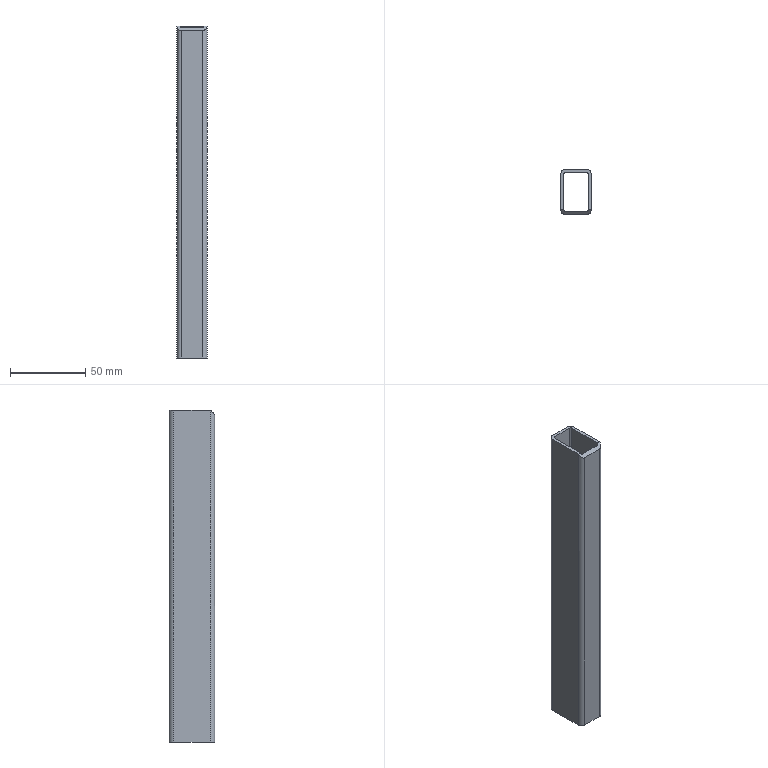Component | SolidWorks | A30x20x2RectangularColdFormedHollowSectionSteel220-1 | 1 solid | 19 faces | box 20 x 30 x 220 mm | volume 38896 mm3 | plane 11 | cylinder 8 | commonest cylinder face diameters 6 x4 2 x4
build123d program:
from build123d import *

# Parameters (mm, degrees)
BOSS_EXTRUDE1_DEPTH     = 220
CUT_EXTRUDE1_DEPTH      = 221.737
CUT_EXTRUDE1_DEPTH_BACK = 221.737


with BuildPart() as part:
    # Sketch1_2 → Boss-Extrude1 (new body)
    with BuildSketch(Plane(origin=(0, 0, 0), x_dir=(0, 0, -1), z_dir=(1, 0, 0))):
        with BuildLine():
            Line((-6.263, 13), (6.263, 13))
            Line((6.263, 13), (7.561, 14.947))
            ThreePointArc((7.561, 14.947), (7.282, 14.987), (7, 15))
            Line((7, 15), (-7, 15))
            ThreePointArc((-7, 15), (-7.282, 14.987), (-7.561, 14.947))
            Line((-7.561, 14.947), (-6.263, 13))
        make_face()
        with BuildLine():
            Line((-10, -11.394), (-8, -8.394))
            Line((-8, -8.394), (-8, 12))
            ThreePointArc((-8, 12), (-7.707, 12.707), (-7, 13))
            Line((-7, 13), (-6.263, 13))
            Line((-6.263, 13), (-7.561, 14.947))
            ThreePointArc((-7.561, 14.947), (-9.311, 13.913), (-10, 12))
            Line((-10, 12), (-10, -11.394))
        make_face()
        with BuildLine():
            Line((8, 12), (8, -8.394))
            Line((8, -8.394), (10, -11.394))
            Line((10, -11.394), (10, 12))
            ThreePointArc((10, 12), (9.311, 13.913), (7.561, 14.947))
            Line((7.561, 14.947), (6.263, 13))
            Line((6.263, 13), (7, 13))
            ThreePointArc((7, 13), (7.707, 12.707), (8, 12))
        make_face()
        with BuildLine():
            Line((7, -13), (-7, -13))
            ThreePointArc((-7, -13), (-7.707, -12.707), (-8, -12))
            Line((-8, -12), (-8, -8.394))
            Line((-8, -8.394), (-10, -11.394))
            Line((-10, -11.394), (-10, -12))
            ThreePointArc((-10, -12), (-9.121, -14.121), (-7, -15))
            Line((-7, -15), (7, -15))
            ThreePointArc((7, -15), (9.121, -14.121), (10, -12))
            Line((10, -12), (10, -11.394))
            Line((10, -11.394), (8, -8.394))
            Line((8, -8.394), (8, -12))
            ThreePointArc((8, -12), (7.707, -12.707), (7, -13))
        make_face()
    extrude(amount=BOSS_EXTRUDE1_DEPTH)

    # Sketch1 → Cut-Extrude1 (cut, two sides: drawn at the far end of the back side and taken through both)
    with BuildSketch(Plane.XY.offset(-CUT_EXTRUDE1_DEPTH_BACK)):
        Polygon((221, 11), (221, 16), (216, 16), align=None)
    extrude(amount=CUT_EXTRUDE1_DEPTH + CUT_EXTRUDE1_DEPTH_BACK, mode=Mode.SUBTRACT)


solid = part.part

# Placed as in the assembly
solid = solid.moved(Location((-452.371, -1060.9, 193), (180, 90, 0)))
STEP:
#1=COLOUR_RGB('',0.7922,0.8196,0.9333);
#2=FILL_AREA_STYLE_COLOUR('',#1);
#3=FILL_AREA_STYLE('',(#2));
#4=SURFACE_STYLE_FILL_AREA(#3);
#5=SURFACE_SIDE_STYLE('',(#4));
#6=SURFACE_STYLE_USAGE(.BOTH.,#5);
#7=PRESENTATION_STYLE_ASSIGNMENT((#6));
#8=CARTESIAN_POINT('',(-17.534,-42.358,16.142));
#9=VERTEX_POINT('',#8);
#10=CARTESIAN_POINT('',(-17.416,-42.24,16.26));
#11=VERTEX_POINT('',#10);
#12=CARTESIAN_POINT('',(-17.534,-42.358,16.142));
#13=CARTESIAN_POINT('',(-17.465,-42.358,16.142));
#14=CARTESIAN_POINT('',(-17.416,-42.309,16.191));
#15=CARTESIAN_POINT('',(-17.416,-42.24,16.26));
#16=(BOUNDED_CURVE()B_SPLINE_CURVE(3,(#12,#13,#14,#15),.UNSPECIFIED.,.F.,.T.)B_SPLINE_CURVE_WITH_KNOTS((4,4),(0.,1.571),.UNSPECIFIED.)CURVE()GEOMETRIC_REPRESENTATION_ITEM()RATIONAL_B_SPLINE_CURVE((1.,0.8047,0.8047,1.))REPRESENTATION_ITEM(''));
#17=EDGE_CURVE('',#9,#11,#16,.T.);
#18=ORIENTED_EDGE('',*,*,#17,.F.);
#19=CARTESIAN_POINT('',(-17.534,-42.358,7.598));
#20=VERTEX_POINT('',#19);
#21=CARTESIAN_POINT('',(-17.534,-42.358,16.26));
#22=DIRECTION('',(0.,0.,-1.));
#23=VECTOR('',#22,39.37);
#24=LINE('',#21,#23);
#25=EDGE_CURVE('',#9,#20,#24,.T.);
#26=ORIENTED_EDGE('',*,*,#25,.T.);
#27=CARTESIAN_POINT('',(-17.416,-42.24,7.598));
#28=VERTEX_POINT('',#27);
#29=CARTESIAN_POINT('',(-17.534,-42.24,7.598));
#30=DIRECTION('',(0.,0.,-1.));
#31=DIRECTION('',(-1.,0.,0.));
#32=AXIS2_PLACEMENT_3D('',#29,#30,#31);
#33=CIRCLE('',#32,0.1181);
#34=EDGE_CURVE('',#28,#20,#33,.T.);
#35=ORIENTED_EDGE('',*,*,#34,.F.);
#36=CARTESIAN_POINT('',(-17.416,-42.24,16.26));
#37=DIRECTION('',(0.,0.,-1.));
#38=VECTOR('',#37,39.37);
#39=LINE('',#36,#38);
#40=EDGE_CURVE('',#11,#28,#39,.T.);
#41=ORIENTED_EDGE('',*,*,#40,.F.);
#42=EDGE_LOOP('',(#18,#26,#35,#41));
#43=FACE_OUTER_BOUND('',#42,.T.);
#44=CARTESIAN_POINT('',(-17.534,-42.24,16.26));
#45=DIRECTION('',(0.,0.,-1.));
#46=DIRECTION('',(1.,0.,0.));
#47=AXIS2_PLACEMENT_3D('',#44,#45,#46);
#48=CYLINDRICAL_SURFACE('',#47,0.1181);
#49=ADVANCED_FACE('',(#43),#48,.T.);
#50=CARTESIAN_POINT('',(-17.416,-41.295,7.598));
#51=VERTEX_POINT('',#50);
#52=CARTESIAN_POINT('',(-17.416,-41.768,7.598));
#53=DIRECTION('',(0.,-1.,-0.));
#54=VECTOR('',#53,39.37);
#55=LINE('',#52,#54);
#56=EDGE_CURVE('',#51,#28,#55,.T.);
#57=ORIENTED_EDGE('',*,*,#56,.F.);
#58=CARTESIAN_POINT('',(-17.416,-41.295,16.26));
#59=VERTEX_POINT('',#58);
#60=CARTESIAN_POINT('',(-17.416,-41.295,16.26));
#61=DIRECTION('',(0.,0.,-1.));
#62=VECTOR('',#61,39.37);
#63=LINE('',#60,#62);
#64=EDGE_CURVE('',#59,#51,#63,.T.);
#65=ORIENTED_EDGE('',*,*,#64,.F.);
#66=CARTESIAN_POINT('',(-17.416,-41.768,16.26));
#67=DIRECTION('',(0.,-1.,-0.));
#68=VECTOR('',#67,39.37);
#69=LINE('',#66,#68);
#70=EDGE_CURVE('',#59,#11,#69,.T.);
#71=ORIENTED_EDGE('',*,*,#70,.T.);
#72=ORIENTED_EDGE('',*,*,#40,.T.);
#73=EDGE_LOOP('',(#57,#65,#71,#72));
#74=FACE_OUTER_BOUND('',#73,.T.);
#75=CARTESIAN_POINT('',(-17.416,-41.768,16.26));
#76=DIRECTION('',(1.,0.,0.));
#77=DIRECTION('',(-0.,-0.,1.));
#78=AXIS2_PLACEMENT_3D('',#75,#76,#77);
#79=PLANE('',#78);
#80=ADVANCED_FACE('',(#74),#79,.T.);
#81=CARTESIAN_POINT('',(-17.534,-41.177,7.598));
#82=VERTEX_POINT('',#81);
#83=CARTESIAN_POINT('',(-17.534,-41.295,7.598));
#84=DIRECTION('',(0.,0.,-1.));
#85=DIRECTION('',(-1.,0.,0.));
#86=AXIS2_PLACEMENT_3D('',#83,#84,#85);
#87=CIRCLE('',#86,0.1181);
#88=EDGE_CURVE('',#82,#51,#87,.T.);
#89=ORIENTED_EDGE('',*,*,#88,.F.);
#90=CARTESIAN_POINT('',(-17.534,-41.177,16.26));
#91=VERTEX_POINT('',#90);
#92=CARTESIAN_POINT('',(-17.534,-41.177,16.26));
#93=DIRECTION('',(0.,0.,-1.));
#94=VECTOR('',#93,39.37);
#95=LINE('',#92,#94);
#96=EDGE_CURVE('',#91,#82,#95,.T.);
#97=ORIENTED_EDGE('',*,*,#96,.F.);
#98=CARTESIAN_POINT('',(-17.534,-41.295,16.26));
#99=DIRECTION('',(0.,0.,-1.));
#100=DIRECTION('',(-1.,0.,0.));
#101=AXIS2_PLACEMENT_3D('',#98,#99,#100);
#102=CIRCLE('',#101,0.1181);
#103=EDGE_CURVE('',#91,#59,#102,.T.);
#104=ORIENTED_EDGE('',*,*,#103,.T.);
#105=ORIENTED_EDGE('',*,*,#64,.T.);
#106=EDGE_LOOP('',(#89,#97,#104,#105));
#107=FACE_OUTER_BOUND('',#106,.T.);
#108=CARTESIAN_POINT('',(-17.534,-41.295,16.26));
#109=DIRECTION('',(0.,0.,-1.));
#110=DIRECTION('',(1.,0.,0.));
#111=AXIS2_PLACEMENT_3D('',#108,#109,#110);
#112=CYLINDRICAL_SURFACE('',#111,0.1181);
#113=ADVANCED_FACE('',(#107),#112,.T.);
#114=CARTESIAN_POINT('',(-18.085,-41.177,7.598));
#115=VERTEX_POINT('',#114);
#116=CARTESIAN_POINT('',(-17.81,-41.177,7.598));
#117=DIRECTION('',(-1.,-0.,-0.));
#118=VECTOR('',#117,39.37);
#119=LINE('',#116,#118);
#120=EDGE_CURVE('',#82,#115,#119,.T.);
#121=ORIENTED_EDGE('',*,*,#120,.T.);
#122=CARTESIAN_POINT('',(-18.085,-41.177,16.26));
#123=VERTEX_POINT('',#122);
#124=CARTESIAN_POINT('',(-18.085,-41.177,16.26));
#125=DIRECTION('',(0.,0.,-1.));
#126=VECTOR('',#125,39.37);
#127=LINE('',#124,#126);
#128=EDGE_CURVE('',#123,#115,#127,.T.);
#129=ORIENTED_EDGE('',*,*,#128,.F.);
#130=CARTESIAN_POINT('',(-17.81,-41.177,16.26));
#131=DIRECTION('',(-1.,-0.,-0.));
#132=VECTOR('',#131,39.37);
#133=LINE('',#130,#132);
#134=EDGE_CURVE('',#91,#123,#133,.T.);
#135=ORIENTED_EDGE('',*,*,#134,.F.);
#136=ORIENTED_EDGE('',*,*,#96,.T.);
#137=EDGE_LOOP('',(#121,#129,#135,#136));
#138=FACE_OUTER_BOUND('',#137,.T.);
#139=CARTESIAN_POINT('',(-17.81,-41.177,16.26));
#140=DIRECTION('',(0.,-1.,-0.));
#141=DIRECTION('',(1.,0.,0.));
#142=AXIS2_PLACEMENT_3D('',#139,#140,#141);
#143=PLANE('',#142);
#144=ADVANCED_FACE('',(#138),#143,.F.);
#145=CARTESIAN_POINT('',(-18.204,-41.295,7.598));
#146=VERTEX_POINT('',#145);
#147=CARTESIAN_POINT('',(-18.085,-41.295,7.598));
#148=DIRECTION('',(-0.,-0.,1.));
#149=DIRECTION('',(-1.,0.,0.));
#150=AXIS2_PLACEMENT_3D('',#147,#148,#149);
#151=CIRCLE('',#150,0.1181);
#152=EDGE_CURVE('',#115,#146,#151,.T.);
#153=ORIENTED_EDGE('',*,*,#152,.T.);
#154=CARTESIAN_POINT('',(-18.204,-41.295,16.26));
#155=VERTEX_POINT('',#154);
#156=CARTESIAN_POINT('',(-18.204,-41.295,16.26));
#157=DIRECTION('',(0.,0.,-1.));
#158=VECTOR('',#157,39.37);
#159=LINE('',#156,#158);
#160=EDGE_CURVE('',#155,#146,#159,.T.);
#161=ORIENTED_EDGE('',*,*,#160,.F.);
#162=CARTESIAN_POINT('',(-18.085,-41.295,16.26));
#163=DIRECTION('',(-0.,-0.,1.));
#164=DIRECTION('',(-1.,0.,0.));
#165=AXIS2_PLACEMENT_3D('',#162,#163,#164);
#166=CIRCLE('',#165,0.1181);
#167=EDGE_CURVE('',#123,#155,#166,.T.);
#168=ORIENTED_EDGE('',*,*,#167,.F.);
#169=ORIENTED_EDGE('',*,*,#128,.T.);
#170=EDGE_LOOP('',(#153,#161,#168,#169));
#171=FACE_OUTER_BOUND('',#170,.T.);
#172=CARTESIAN_POINT('',(-18.085,-41.295,16.26));
#173=DIRECTION('',(0.,0.,-1.));
#174=DIRECTION('',(1.,0.,0.));
#175=AXIS2_PLACEMENT_3D('',#172,#173,#174);
#176=CYLINDRICAL_SURFACE('',#175,0.1181);
#177=ADVANCED_FACE('',(#171),#176,.T.);
#178=CARTESIAN_POINT('',(-18.204,-42.24,7.598));
#179=VERTEX_POINT('',#178);
#180=CARTESIAN_POINT('',(-18.204,-41.768,7.598));
#181=DIRECTION('',(0.,-1.,-0.));
#182=VECTOR('',#181,39.37);
#183=LINE('',#180,#182);
#184=EDGE_CURVE('',#146,#179,#183,.T.);
#185=ORIENTED_EDGE('',*,*,#184,.T.);
#186=CARTESIAN_POINT('',(-18.204,-42.24,16.26));
#187=VERTEX_POINT('',#186);
#188=CARTESIAN_POINT('',(-18.204,-42.24,16.26));
#189=DIRECTION('',(0.,0.,-1.));
#190=VECTOR('',#189,39.37);
#191=LINE('',#188,#190);
#192=EDGE_CURVE('',#187,#179,#191,.T.);
#193=ORIENTED_EDGE('',*,*,#192,.F.);
#194=CARTESIAN_POINT('',(-18.204,-41.768,16.26));
#195=DIRECTION('',(0.,-1.,-0.));
#196=VECTOR('',#195,39.37);
#197=LINE('',#194,#196);
#198=EDGE_CURVE('',#155,#187,#197,.T.);
#199=ORIENTED_EDGE('',*,*,#198,.F.);
#200=ORIENTED_EDGE('',*,*,#160,.T.);
#201=EDGE_LOOP('',(#185,#193,#199,#200));
#202=FACE_OUTER_BOUND('',#201,.T.);
#203=CARTESIAN_POINT('',(-18.204,-41.768,16.26));
#204=DIRECTION('',(1.,0.,0.));
#205=DIRECTION('',(-0.,-0.,1.));
#206=AXIS2_PLACEMENT_3D('',#203,#204,#205);
#207=PLANE('',#206);
#208=ADVANCED_FACE('',(#202),#207,.F.);
#209=CARTESIAN_POINT('',(-18.085,-42.358,16.142));
#210=VERTEX_POINT('',#209);
#211=CARTESIAN_POINT('',(-18.204,-42.24,16.26));
#212=CARTESIAN_POINT('',(-18.204,-42.309,16.191));
#213=CARTESIAN_POINT('',(-18.155,-42.358,16.142));
#214=CARTESIAN_POINT('',(-18.085,-42.358,16.142));
#215=(BOUNDED_CURVE()B_SPLINE_CURVE(3,(#211,#212,#213,#214),.UNSPECIFIED.,.F.,.T.)B_SPLINE_CURVE_WITH_KNOTS((4,4),(4.712,6.283),.UNSPECIFIED.)CURVE()GEOMETRIC_REPRESENTATION_ITEM()RATIONAL_B_SPLINE_CURVE((1.,0.8047,0.8047,1.))REPRESENTATION_ITEM(''));
#216=EDGE_CURVE('',#187,#210,#215,.T.);
#217=ORIENTED_EDGE('',*,*,#216,.F.);
#218=ORIENTED_EDGE('',*,*,#192,.T.);
#219=CARTESIAN_POINT('',(-18.085,-42.358,7.598));
#220=VERTEX_POINT('',#219);
#221=CARTESIAN_POINT('',(-18.085,-42.24,7.598));
#222=DIRECTION('',(0.,0.,-1.));
#223=DIRECTION('',(-1.,0.,0.));
#224=AXIS2_PLACEMENT_3D('',#221,#222,#223);
#225=CIRCLE('',#224,0.1181);
#226=EDGE_CURVE('',#220,#179,#225,.T.);
#227=ORIENTED_EDGE('',*,*,#226,.F.);
#228=CARTESIAN_POINT('',(-18.085,-42.358,16.26));
#229=DIRECTION('',(0.,0.,-1.));
#230=VECTOR('',#229,39.37);
#231=LINE('',#228,#230);
#232=EDGE_CURVE('',#210,#220,#231,.T.);
#233=ORIENTED_EDGE('',*,*,#232,.F.);
#234=EDGE_LOOP('',(#217,#218,#227,#233));
#235=FACE_OUTER_BOUND('',#234,.T.);
#236=CARTESIAN_POINT('',(-18.085,-42.24,16.26));
#237=DIRECTION('',(0.,0.,-1.));
#238=DIRECTION('',(1.,0.,0.));
#239=AXIS2_PLACEMENT_3D('',#236,#237,#238);
#240=CYLINDRICAL_SURFACE('',#239,0.1181);
#241=ADVANCED_FACE('',(#235),#240,.T.);
#242=CARTESIAN_POINT('',(-17.534,-41.256,7.598));
#243=VERTEX_POINT('',#242);
#244=CARTESIAN_POINT('',(-17.495,-41.295,7.598));
#245=VERTEX_POINT('',#244);
#246=CARTESIAN_POINT('',(-17.534,-41.295,7.598));
#247=DIRECTION('',(0.,0.,-1.));
#248=DIRECTION('',(-1.,0.,0.));
#249=AXIS2_PLACEMENT_3D('',#246,#247,#248);
#250=CIRCLE('',#249,0.03937);
#251=EDGE_CURVE('',#243,#245,#250,.T.);
#252=ORIENTED_EDGE('',*,*,#251,.T.);
#253=CARTESIAN_POINT('',(-17.495,-41.295,16.26));
#254=VERTEX_POINT('',#253);
#255=CARTESIAN_POINT('',(-17.495,-41.295,16.26));
#256=DIRECTION('',(0.,0.,-1.));
#257=VECTOR('',#256,39.37);
#258=LINE('',#255,#257);
#259=EDGE_CURVE('',#254,#245,#258,.T.);
#260=ORIENTED_EDGE('',*,*,#259,.F.);
#261=CARTESIAN_POINT('',(-17.534,-41.256,16.26));
#262=VERTEX_POINT('',#261);
#263=CARTESIAN_POINT('',(-17.534,-41.295,16.26));
#264=DIRECTION('',(0.,0.,-1.));
#265=DIRECTION('',(-1.,0.,0.));
#266=AXIS2_PLACEMENT_3D('',#263,#264,#265);
#267=CIRCLE('',#266,0.03937);
#268=EDGE_CURVE('',#262,#254,#267,.T.);
#269=ORIENTED_EDGE('',*,*,#268,.F.);
#270=CARTESIAN_POINT('',(-17.534,-41.256,16.26));
#271=DIRECTION('',(0.,0.,-1.));
#272=VECTOR('',#271,39.37);
#273=LINE('',#270,#272);
#274=EDGE_CURVE('',#262,#243,#273,.T.);
#275=ORIENTED_EDGE('',*,*,#274,.T.);
#276=EDGE_LOOP('',(#252,#260,#269,#275));
#277=FACE_OUTER_BOUND('',#276,.T.);
#278=CARTESIAN_POINT('',(-17.534,-41.295,16.26));
#279=DIRECTION('',(0.,0.,-1.));
#280=DIRECTION('',(1.,0.,0.));
#281=AXIS2_PLACEMENT_3D('',#278,#279,#280);
#282=CYLINDRICAL_SURFACE('',#281,0.03937);
#283=ADVANCED_FACE('',(#277),#282,.F.);
#284=CARTESIAN_POINT('',(-17.495,-42.24,7.598));
#285=VERTEX_POINT('',#284);
#286=CARTESIAN_POINT('',(-17.495,-41.768,7.598));
#287=DIRECTION('',(0.,-1.,-0.));
#288=VECTOR('',#287,39.37);
#289=LINE('',#286,#288);
#290=EDGE_CURVE('',#245,#285,#289,.T.);
#291=ORIENTED_EDGE('',*,*,#290,.T.);
#292=CARTESIAN_POINT('',(-17.495,-42.24,16.26));
#293=VERTEX_POINT('',#292);
#294=CARTESIAN_POINT('',(-17.495,-42.24,16.26));
#295=DIRECTION('',(0.,0.,-1.));
#296=VECTOR('',#295,39.37);
#297=LINE('',#294,#296);
#298=EDGE_CURVE('',#293,#285,#297,.T.);
#299=ORIENTED_EDGE('',*,*,#298,.F.);
#300=CARTESIAN_POINT('',(-17.495,-41.768,16.26));
#301=DIRECTION('',(0.,-1.,-0.));
#302=VECTOR('',#301,39.37);
#303=LINE('',#300,#302);
#304=EDGE_CURVE('',#254,#293,#303,.T.);
#305=ORIENTED_EDGE('',*,*,#304,.F.);
#306=ORIENTED_EDGE('',*,*,#259,.T.);
#307=EDGE_LOOP('',(#291,#299,#305,#306));
#308=FACE_OUTER_BOUND('',#307,.T.);
#309=CARTESIAN_POINT('',(-17.495,-41.768,16.26));
#310=DIRECTION('',(1.,0.,0.));
#311=DIRECTION('',(-0.,-0.,1.));
#312=AXIS2_PLACEMENT_3D('',#309,#310,#311);
#313=PLANE('',#312);
#314=ADVANCED_FACE('',(#308),#313,.F.);
#315=CARTESIAN_POINT('',(-17.534,-42.28,16.22));
#316=VERTEX_POINT('',#315);
#317=CARTESIAN_POINT('',(-17.534,-42.28,7.598));
#318=VERTEX_POINT('',#317);
#319=CARTESIAN_POINT('',(-17.534,-42.28,16.26));
#320=DIRECTION('',(0.,0.,-1.));
#321=VECTOR('',#320,39.37);
#322=LINE('',#319,#321);
#323=EDGE_CURVE('',#316,#318,#322,.T.);
#324=ORIENTED_EDGE('',*,*,#323,.F.);
#325=CARTESIAN_POINT('',(-17.534,-42.28,16.22));
#326=CARTESIAN_POINT('',(-17.511,-42.28,16.22));
#327=CARTESIAN_POINT('',(-17.495,-42.263,16.237));
#328=CARTESIAN_POINT('',(-17.495,-42.24,16.26));
#329=(BOUNDED_CURVE()B_SPLINE_CURVE(3,(#325,#326,#327,#328),.UNSPECIFIED.,.F.,.T.)B_SPLINE_CURVE_WITH_KNOTS((4,4),(0.,1.571),.UNSPECIFIED.)CURVE()GEOMETRIC_REPRESENTATION_ITEM()RATIONAL_B_SPLINE_CURVE((1.,0.8047,0.8047,1.))REPRESENTATION_ITEM(''));
#330=EDGE_CURVE('',#316,#293,#329,.T.);
#331=ORIENTED_EDGE('',*,*,#330,.T.);
#332=ORIENTED_EDGE('',*,*,#298,.T.);
#333=CARTESIAN_POINT('',(-17.534,-42.24,7.598));
#334=DIRECTION('',(0.,0.,-1.));
#335=DIRECTION('',(-1.,0.,0.));
#336=AXIS2_PLACEMENT_3D('',#333,#334,#335);
#337=CIRCLE('',#336,0.03937);
#338=EDGE_CURVE('',#285,#318,#337,.T.);
#339=ORIENTED_EDGE('',*,*,#338,.T.);
#340=EDGE_LOOP('',(#324,#331,#332,#339));
#341=FACE_OUTER_BOUND('',#340,.T.);
#342=CARTESIAN_POINT('',(-17.534,-42.24,16.26));
#343=DIRECTION('',(0.,0.,-1.));
#344=DIRECTION('',(1.,0.,0.));
#345=AXIS2_PLACEMENT_3D('',#342,#343,#344);
#346=CYLINDRICAL_SURFACE('',#345,0.03937);
#347=ADVANCED_FACE('',(#341),#346,.F.);
#348=CARTESIAN_POINT('',(-18.085,-42.28,16.22));
#349=VERTEX_POINT('',#348);
#350=CARTESIAN_POINT('',(-18.085,-42.28,7.598));
#351=VERTEX_POINT('',#350);
#352=CARTESIAN_POINT('',(-18.085,-42.28,16.26));
#353=DIRECTION('',(0.,0.,-1.));
#354=VECTOR('',#353,39.37);
#355=LINE('',#352,#354);
#356=EDGE_CURVE('',#349,#351,#355,.T.);
#357=ORIENTED_EDGE('',*,*,#356,.F.);
#358=CARTESIAN_POINT('',(-17.81,-42.28,16.22));
#359=DIRECTION('',(1.,0.,0.));
#360=VECTOR('',#359,39.37);
#361=LINE('',#358,#360);
#362=EDGE_CURVE('',#349,#316,#361,.T.);
#363=ORIENTED_EDGE('',*,*,#362,.T.);
#364=ORIENTED_EDGE('',*,*,#323,.T.);
#365=CARTESIAN_POINT('',(-17.81,-42.28,7.598));
#366=DIRECTION('',(-1.,-0.,-0.));
#367=VECTOR('',#366,39.37);
#368=LINE('',#365,#367);
#369=EDGE_CURVE('',#318,#351,#368,.T.);
#370=ORIENTED_EDGE('',*,*,#369,.T.);
#371=EDGE_LOOP('',(#357,#363,#364,#370));
#372=FACE_OUTER_BOUND('',#371,.T.);
#373=CARTESIAN_POINT('',(-17.81,-42.28,16.26));
#374=DIRECTION('',(0.,-1.,-0.));
#375=DIRECTION('',(1.,0.,0.));
#376=AXIS2_PLACEMENT_3D('',#373,#374,#375);
#377=PLANE('',#376);
#378=ADVANCED_FACE('',(#372),#377,.F.);
#379=CARTESIAN_POINT('',(-18.125,-42.24,16.26));
#380=VERTEX_POINT('',#379);
#381=CARTESIAN_POINT('',(-18.125,-42.24,7.598));
#382=VERTEX_POINT('',#381);
#383=CARTESIAN_POINT('',(-18.125,-42.24,16.26));
#384=DIRECTION('',(0.,0.,-1.));
#385=VECTOR('',#384,39.37);
#386=LINE('',#383,#385);
#387=EDGE_CURVE('',#380,#382,#386,.T.);
#388=ORIENTED_EDGE('',*,*,#387,.F.);
#389=CARTESIAN_POINT('',(-18.125,-42.24,16.26));
#390=CARTESIAN_POINT('',(-18.125,-42.263,16.237));
#391=CARTESIAN_POINT('',(-18.109,-42.28,16.22));
#392=CARTESIAN_POINT('',(-18.085,-42.28,16.22));
#393=(BOUNDED_CURVE()B_SPLINE_CURVE(3,(#389,#390,#391,#392),.UNSPECIFIED.,.F.,.T.)B_SPLINE_CURVE_WITH_KNOTS((4,4),(4.712,6.283),.UNSPECIFIED.)CURVE()GEOMETRIC_REPRESENTATION_ITEM()RATIONAL_B_SPLINE_CURVE((1.,0.8047,0.8047,1.))REPRESENTATION_ITEM(''));
#394=EDGE_CURVE('',#380,#349,#393,.T.);
#395=ORIENTED_EDGE('',*,*,#394,.T.);
#396=ORIENTED_EDGE('',*,*,#356,.T.);
#397=CARTESIAN_POINT('',(-18.085,-42.24,7.598));
#398=DIRECTION('',(0.,0.,-1.));
#399=DIRECTION('',(-1.,0.,0.));
#400=AXIS2_PLACEMENT_3D('',#397,#398,#399);
#401=CIRCLE('',#400,0.03937);
#402=EDGE_CURVE('',#351,#382,#401,.T.);
#403=ORIENTED_EDGE('',*,*,#402,.T.);
#404=EDGE_LOOP('',(#388,#395,#396,#403));
#405=FACE_OUTER_BOUND('',#404,.T.);
#406=CARTESIAN_POINT('',(-18.085,-42.24,16.26));
#407=DIRECTION('',(0.,0.,-1.));
#408=DIRECTION('',(1.,0.,0.));
#409=AXIS2_PLACEMENT_3D('',#406,#407,#408);
#410=CYLINDRICAL_SURFACE('',#409,0.03937);
#411=ADVANCED_FACE('',(#405),#410,.F.);
#412=CARTESIAN_POINT('',(-18.125,-41.295,7.598));
#413=VERTEX_POINT('',#412);
#414=CARTESIAN_POINT('',(-18.125,-41.768,7.598));
#415=DIRECTION('',(0.,-1.,-0.));
#416=VECTOR('',#415,39.37);
#417=LINE('',#414,#416);
#418=EDGE_CURVE('',#413,#382,#417,.T.);
#419=ORIENTED_EDGE('',*,*,#418,.F.);
#420=CARTESIAN_POINT('',(-18.125,-41.295,16.26));
#421=VERTEX_POINT('',#420);
#422=CARTESIAN_POINT('',(-18.125,-41.295,16.26));
#423=DIRECTION('',(0.,0.,-1.));
#424=VECTOR('',#423,39.37);
#425=LINE('',#422,#424);
#426=EDGE_CURVE('',#421,#413,#425,.T.);
#427=ORIENTED_EDGE('',*,*,#426,.F.);
#428=CARTESIAN_POINT('',(-18.125,-41.768,16.26));
#429=DIRECTION('',(0.,-1.,-0.));
#430=VECTOR('',#429,39.37);
#431=LINE('',#428,#430);
#432=EDGE_CURVE('',#421,#380,#431,.T.);
#433=ORIENTED_EDGE('',*,*,#432,.T.);
#434=ORIENTED_EDGE('',*,*,#387,.T.);
#435=EDGE_LOOP('',(#419,#427,#433,#434));
#436=FACE_OUTER_BOUND('',#435,.T.);
#437=CARTESIAN_POINT('',(-18.125,-41.768,16.26));
#438=DIRECTION('',(1.,0.,0.));
#439=DIRECTION('',(-0.,-0.,1.));
#440=AXIS2_PLACEMENT_3D('',#437,#438,#439);
#441=PLANE('',#440);
#442=ADVANCED_FACE('',(#436),#441,.T.);
#443=CARTESIAN_POINT('',(-18.085,-41.256,7.598));
#444=VERTEX_POINT('',#443);
#445=CARTESIAN_POINT('',(-18.085,-41.295,7.598));
#446=DIRECTION('',(-0.,-0.,1.));
#447=DIRECTION('',(-1.,0.,0.));
#448=AXIS2_PLACEMENT_3D('',#445,#446,#447);
#449=CIRCLE('',#448,0.03937);
#450=EDGE_CURVE('',#444,#413,#449,.T.);
#451=ORIENTED_EDGE('',*,*,#450,.F.);
#452=CARTESIAN_POINT('',(-18.085,-41.256,16.26));
#453=VERTEX_POINT('',#452);
#454=CARTESIAN_POINT('',(-18.085,-41.256,16.26));
#455=DIRECTION('',(0.,0.,-1.));
#456=VECTOR('',#455,39.37);
#457=LINE('',#454,#456);
#458=EDGE_CURVE('',#453,#444,#457,.T.);
#459=ORIENTED_EDGE('',*,*,#458,.F.);
#460=CARTESIAN_POINT('',(-18.085,-41.295,16.26));
#461=DIRECTION('',(-0.,-0.,1.));
#462=DIRECTION('',(-1.,0.,0.));
#463=AXIS2_PLACEMENT_3D('',#460,#461,#462);
#464=CIRCLE('',#463,0.03937);
#465=EDGE_CURVE('',#453,#421,#464,.T.);
#466=ORIENTED_EDGE('',*,*,#465,.T.);
#467=ORIENTED_EDGE('',*,*,#426,.T.);
#468=EDGE_LOOP('',(#451,#459,#466,#467));
#469=FACE_OUTER_BOUND('',#468,.T.);
#470=CARTESIAN_POINT('',(-18.085,-41.295,16.26));
#471=DIRECTION('',(0.,0.,-1.));
#472=DIRECTION('',(1.,0.,0.));
#473=AXIS2_PLACEMENT_3D('',#470,#471,#472);
#474=CYLINDRICAL_SURFACE('',#473,0.03937);
#475=ADVANCED_FACE('',(#469),#474,.F.);
#476=CARTESIAN_POINT('',(-17.81,-41.256,7.598));
#477=DIRECTION('',(-1.,-0.,-0.));
#478=VECTOR('',#477,39.37);
#479=LINE('',#476,#478);
#480=EDGE_CURVE('',#243,#444,#479,.T.);
#481=ORIENTED_EDGE('',*,*,#480,.F.);
#482=ORIENTED_EDGE('',*,*,#274,.F.);
#483=CARTESIAN_POINT('',(-17.81,-41.256,16.26));
#484=DIRECTION('',(-1.,-0.,-0.));
#485=VECTOR('',#484,39.37);
#486=LINE('',#483,#485);
#487=EDGE_CURVE('',#262,#453,#486,.T.);
#488=ORIENTED_EDGE('',*,*,#487,.T.);
#489=ORIENTED_EDGE('',*,*,#458,.T.);
#490=EDGE_LOOP('',(#481,#482,#488,#489));
#491=FACE_OUTER_BOUND('',#490,.T.);
#492=CARTESIAN_POINT('',(-17.81,-41.256,16.26));
#493=DIRECTION('',(0.,-1.,-0.));
#494=DIRECTION('',(1.,0.,0.));
#495=AXIS2_PLACEMENT_3D('',#492,#493,#494);
#496=PLANE('',#495);
#497=ADVANCED_FACE('',(#491),#496,.T.);
#498=CARTESIAN_POINT('',(-17.81,-42.358,16.142));
#499=DIRECTION('',(1.,0.,0.));
#500=VECTOR('',#499,39.37);
#501=LINE('',#498,#500);
#502=EDGE_CURVE('',#210,#9,#501,.T.);
#503=ORIENTED_EDGE('',*,*,#502,.F.);
#504=ORIENTED_EDGE('',*,*,#232,.T.);
#505=CARTESIAN_POINT('',(-17.81,-42.358,7.598));
#506=DIRECTION('',(-1.,-0.,-0.));
#507=VECTOR('',#506,39.37);
#508=LINE('',#505,#507);
#509=EDGE_CURVE('',#20,#220,#508,.T.);
#510=ORIENTED_EDGE('',*,*,#509,.F.);
#511=ORIENTED_EDGE('',*,*,#25,.F.);
#512=EDGE_LOOP('',(#503,#504,#510,#511));
#513=FACE_OUTER_BOUND('',#512,.T.);
#514=CARTESIAN_POINT('',(-17.81,-42.358,16.26));
#515=DIRECTION('',(0.,-1.,-0.));
#516=DIRECTION('',(1.,0.,0.));
#517=AXIS2_PLACEMENT_3D('',#514,#515,#516);
#518=PLANE('',#517);
#519=ADVANCED_FACE('',(#513),#518,.T.);
#520=CARTESIAN_POINT('',(-17.81,-42.24,16.26));
#521=DIRECTION('',(-1.,-0.,-0.));
#522=VECTOR('',#521,39.37);
#523=LINE('',#520,#522);
#524=EDGE_CURVE('',#11,#293,#523,.T.);
#525=ORIENTED_EDGE('',*,*,#524,.F.);
#526=ORIENTED_EDGE('',*,*,#70,.F.);
#527=ORIENTED_EDGE('',*,*,#103,.F.);
#528=ORIENTED_EDGE('',*,*,#134,.T.);
#529=ORIENTED_EDGE('',*,*,#167,.T.);
#530=ORIENTED_EDGE('',*,*,#198,.T.);
#531=CARTESIAN_POINT('',(-17.81,-42.24,16.26));
#532=DIRECTION('',(-1.,-0.,-0.));
#533=VECTOR('',#532,39.37);
#534=LINE('',#531,#533);
#535=EDGE_CURVE('',#380,#187,#534,.T.);
#536=ORIENTED_EDGE('',*,*,#535,.F.);
#537=ORIENTED_EDGE('',*,*,#432,.F.);
#538=ORIENTED_EDGE('',*,*,#465,.F.);
#539=ORIENTED_EDGE('',*,*,#487,.F.);
#540=ORIENTED_EDGE('',*,*,#268,.T.);
#541=ORIENTED_EDGE('',*,*,#304,.T.);
#542=EDGE_LOOP('',(#525,#526,#527,#528,#529,#530,#536,#537,#538,#539,#540,#541));
#543=FACE_OUTER_BOUND('',#542,.T.);
#544=CARTESIAN_POINT('',(-17.81,-41.768,16.26));
#545=DIRECTION('',(-0.,-0.,1.));
#546=DIRECTION('',(-1.,-0.,-0.));
#547=AXIS2_PLACEMENT_3D('',#544,#545,#546);
#548=PLANE('',#547);
#549=ADVANCED_FACE('',(#543),#548,.T.);
#550=ORIENTED_EDGE('',*,*,#251,.F.);
#551=ORIENTED_EDGE('',*,*,#480,.T.);
#552=ORIENTED_EDGE('',*,*,#450,.T.);
#553=ORIENTED_EDGE('',*,*,#418,.T.);
#554=ORIENTED_EDGE('',*,*,#402,.F.);
#555=ORIENTED_EDGE('',*,*,#369,.F.);
#556=ORIENTED_EDGE('',*,*,#338,.F.);
#557=ORIENTED_EDGE('',*,*,#290,.F.);
#558=EDGE_LOOP('',(#550,#551,#552,#553,#554,#555,#556,#557));
#559=FACE_BOUND('',#558,.T.);
#560=ORIENTED_EDGE('',*,*,#34,.T.);
#561=ORIENTED_EDGE('',*,*,#509,.T.);
#562=ORIENTED_EDGE('',*,*,#226,.T.);
#563=ORIENTED_EDGE('',*,*,#184,.F.);
#564=ORIENTED_EDGE('',*,*,#152,.F.);
#565=ORIENTED_EDGE('',*,*,#120,.F.);
#566=ORIENTED_EDGE('',*,*,#88,.T.);
#567=ORIENTED_EDGE('',*,*,#56,.T.);
#568=EDGE_LOOP('',(#560,#561,#562,#563,#564,#565,#566,#567));
#569=FACE_OUTER_BOUND('',#568,.T.);
#570=CARTESIAN_POINT('',(-17.81,-41.768,7.598));
#571=DIRECTION('',(-0.,-0.,1.));
#572=DIRECTION('',(-1.,-0.,-0.));
#573=AXIS2_PLACEMENT_3D('',#570,#571,#572);
#574=PLANE('',#573);
#575=ADVANCED_FACE('',(#559,#569),#574,.F.);
#576=ORIENTED_EDGE('',*,*,#17,.T.);
#577=ORIENTED_EDGE('',*,*,#524,.T.);
#578=ORIENTED_EDGE('',*,*,#330,.F.);
#579=ORIENTED_EDGE('',*,*,#362,.F.);
#580=ORIENTED_EDGE('',*,*,#394,.F.);
#581=ORIENTED_EDGE('',*,*,#535,.T.);
#582=ORIENTED_EDGE('',*,*,#216,.T.);
#583=ORIENTED_EDGE('',*,*,#502,.T.);
#584=EDGE_LOOP('',(#576,#577,#578,#579,#580,#581,#582,#583));
#585=FACE_OUTER_BOUND('',#584,.T.);
#586=CARTESIAN_POINT('',(-18.204,-42.398,16.102));
#587=DIRECTION('',(-0.,0.7071,-0.7071));
#588=DIRECTION('',(-0.,0.7071,0.7071));
#589=AXIS2_PLACEMENT_3D('',#586,#587,#588);
#590=PLANE('',#589);
#591=ADVANCED_FACE('',(#585),#590,.F.);
#592=CLOSED_SHELL('',(#49,#80,#113,#144,#177,#208,#241,#283,#314,#347,#378,#411,#442,#475,#497,#519,#549,#575,#591));
#593=MANIFOLD_SOLID_BREP('',#592);
#594=STYLED_ITEM('',(#7),#593);
#595=(LENGTH_UNIT()NAMED_UNIT(*)SI_UNIT($,.METRE.));
#596=LENGTH_MEASURE_WITH_UNIT(LENGTH_MEASURE(0.0254),#595);
#597=DIMENSIONAL_EXPONENTS(1.,0.,0.,0.,0.,0.,0.);
#598=(CONVERSION_BASED_UNIT('',#596)LENGTH_UNIT()NAMED_UNIT(#597));
#599=UNCERTAINTY_MEASURE_WITH_UNIT(LENGTH_MEASURE(0.00001),#598,'','');
#600=(NAMED_UNIT(*)PLANE_ANGLE_UNIT()SI_UNIT($,.RADIAN.));
#601=(NAMED_UNIT(*)SI_UNIT($,.STERADIAN.)SOLID_ANGLE_UNIT());
#602=(GEOMETRIC_REPRESENTATION_CONTEXT(3)GLOBAL_UNCERTAINTY_ASSIGNED_CONTEXT((#599))GLOBAL_UNIT_ASSIGNED_CONTEXT((#598,#600,#601))REPRESENTATION_CONTEXT('',''));
#603=MECHANICAL_DESIGN_GEOMETRIC_PRESENTATION_REPRESENTATION('',(#594),#602);
#604=PRESENTATION_LAYER_ASSIGNMENT('','',(#594));
#605=CARTESIAN_POINT('',(0.,0.,0.));
#606=DIRECTION('',(0.,0.,1.));
#607=DIRECTION('',(1.,0.,0.));
#608=AXIS2_PLACEMENT_3D('',#605,#606,#607);
#609=(LENGTH_UNIT()NAMED_UNIT(*)SI_UNIT($,.METRE.));
#610=LENGTH_MEASURE_WITH_UNIT(LENGTH_MEASURE(0.0254),#609);
#611=DIMENSIONAL_EXPONENTS(1.,0.,0.,0.,0.,0.,0.);
#612=(CONVERSION_BASED_UNIT('',#610)LENGTH_UNIT()NAMED_UNIT(#611));
#613=UNCERTAINTY_MEASURE_WITH_UNIT(LENGTH_MEASURE(0.00001),#612,'','');
#614=(NAMED_UNIT(*)PLANE_ANGLE_UNIT()SI_UNIT($,.RADIAN.));
#615=(NAMED_UNIT(*)SI_UNIT($,.STERADIAN.)SOLID_ANGLE_UNIT());
#616=(GEOMETRIC_REPRESENTATION_CONTEXT(3)GLOBAL_UNCERTAINTY_ASSIGNED_CONTEXT((#613))GLOBAL_UNIT_ASSIGNED_CONTEXT((#612,#614,#615))REPRESENTATION_CONTEXT('',''));
#617=ADVANCED_BREP_SHAPE_REPRESENTATION('',(#593,#608),#616);